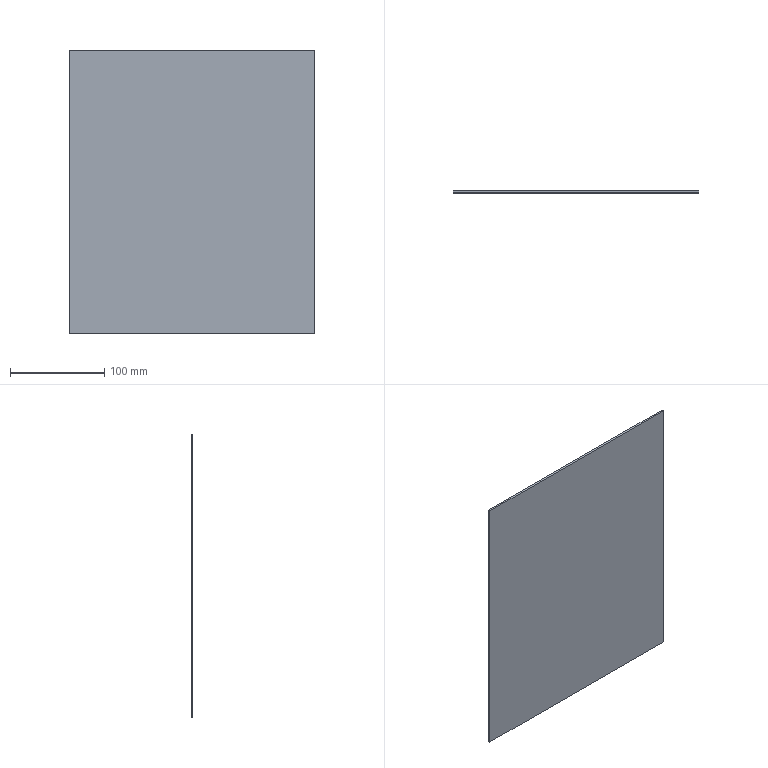Component | SolidWorks | SL010-Material-1 | 1 solid | 16 faces | box 260 x 2 x 300 mm | volume 155979 mm3 | plane 16
build123d program:
from build123d import *

# Parameters (mm, degrees)
SKETCH1_W           = 300
SKETCH1_H           = 260
BOSS_EXTRUDE1_DEPTH = 2
SKETCH2_W           = 284
SKETCH2_H           = 244
SKETCH2_W_2         = 283.6
SKETCH2_H_2         = 243.6
CUT_EXTRUDE1_DEPTH  = 0.1


with BuildPart() as part:
    # Sketch1 → Boss-Extrude1 (new body)
    with BuildSketch(Plane(origin=(0, 0, 0), x_dir=(1, 0, 0), z_dir=(0, 1, 0))):
        Rectangle(SKETCH1_W, SKETCH1_H)
    extrude(amount=BOSS_EXTRUDE1_DEPTH)

    # Sketch2 → Cut-Extrude1 (cut)
    with BuildSketch(Plane(origin=(0, 2, 0), x_dir=(1, 0, 0), z_dir=(0, 1, 0))):
        Rectangle(SKETCH2_W, SKETCH2_H)
        Rectangle(SKETCH2_W_2, SKETCH2_H_2, mode=Mode.SUBTRACT)
    extrude(amount=-CUT_EXTRUDE1_DEPTH, mode=Mode.SUBTRACT)


solid = part.part

# Placed as in the assembly
solid = solid.moved(Location((-535, -109.904, -487.035), (0, 90, 0)))
STEP:
#1=CARTESIAN_POINT('',(-15.945,-4.327,-25.08));
#2=VERTEX_POINT('',#1);
#3=CARTESIAN_POINT('',(-26.181,-4.327,-25.08));
#4=VERTEX_POINT('',#3);
#5=CARTESIAN_POINT('',(-26.181,-4.327,-25.08));
#6=DIRECTION('',(-1.,0.,0.));
#7=VECTOR('',#6,39.37);
#8=LINE('',#5,#7);
#9=EDGE_CURVE('',#2,#4,#8,.T.);
#10=ORIENTED_EDGE('',*,*,#9,.T.);
#11=CARTESIAN_POINT('',(-26.181,-4.248,-25.08));
#12=VERTEX_POINT('',#11);
#13=CARTESIAN_POINT('',(-26.181,-4.248,-25.08));
#14=DIRECTION('',(-0.,-1.,-0.));
#15=VECTOR('',#14,39.37);
#16=LINE('',#13,#15);
#17=EDGE_CURVE('',#12,#4,#16,.T.);
#18=ORIENTED_EDGE('',*,*,#17,.F.);
#19=CARTESIAN_POINT('',(-15.945,-4.248,-25.08));
#20=VERTEX_POINT('',#19);
#21=CARTESIAN_POINT('',(-26.181,-4.248,-25.08));
#22=DIRECTION('',(-1.,0.,0.));
#23=VECTOR('',#22,39.37);
#24=LINE('',#21,#23);
#25=EDGE_CURVE('',#20,#12,#24,.T.);
#26=ORIENTED_EDGE('',*,*,#25,.F.);
#27=CARTESIAN_POINT('',(-15.945,-4.248,-25.08));
#28=DIRECTION('',(-0.,-1.,-0.));
#29=VECTOR('',#28,39.37);
#30=LINE('',#27,#29);
#31=EDGE_CURVE('',#20,#2,#30,.T.);
#32=ORIENTED_EDGE('',*,*,#31,.T.);
#33=EDGE_LOOP('',(#10,#18,#26,#32));
#34=FACE_OUTER_BOUND('',#33,.T.);
#35=CARTESIAN_POINT('',(-26.181,-4.248,-25.08));
#36=DIRECTION('',(0.,-0.,1.));
#37=DIRECTION('',(1.,-0.,-0.));
#38=AXIS2_PLACEMENT_3D('',#35,#36,#37);
#39=PLANE('',#38);
#40=ADVANCED_FACE('',(#34),#39,.F.);
#41=CARTESIAN_POINT('',(-26.181,-4.327,-13.269));
#42=VERTEX_POINT('',#41);
#43=CARTESIAN_POINT('',(-26.181,-4.327,-13.269));
#44=DIRECTION('',(0.,-0.,1.));
#45=VECTOR('',#44,39.37);
#46=LINE('',#43,#45);
#47=EDGE_CURVE('',#4,#42,#46,.T.);
#48=ORIENTED_EDGE('',*,*,#47,.T.);
#49=CARTESIAN_POINT('',(-26.181,-4.248,-13.269));
#50=VERTEX_POINT('',#49);
#51=CARTESIAN_POINT('',(-26.181,-4.248,-13.269));
#52=DIRECTION('',(-0.,-1.,-0.));
#53=VECTOR('',#52,39.37);
#54=LINE('',#51,#53);
#55=EDGE_CURVE('',#50,#42,#54,.T.);
#56=ORIENTED_EDGE('',*,*,#55,.F.);
#57=CARTESIAN_POINT('',(-26.181,-4.248,-13.269));
#58=DIRECTION('',(0.,-0.,1.));
#59=VECTOR('',#58,39.37);
#60=LINE('',#57,#59);
#61=EDGE_CURVE('',#12,#50,#60,.T.);
#62=ORIENTED_EDGE('',*,*,#61,.F.);
#63=ORIENTED_EDGE('',*,*,#17,.T.);
#64=EDGE_LOOP('',(#48,#56,#62,#63));
#65=FACE_OUTER_BOUND('',#64,.T.);
#66=CARTESIAN_POINT('',(-26.181,-4.248,-13.269));
#67=DIRECTION('',(1.,-0.,-0.));
#68=DIRECTION('',(-0.,0.,-1.));
#69=AXIS2_PLACEMENT_3D('',#66,#67,#68);
#70=PLANE('',#69);
#71=ADVANCED_FACE('',(#65),#70,.F.);
#72=CARTESIAN_POINT('',(-15.945,-4.327,-13.269));
#73=VERTEX_POINT('',#72);
#74=CARTESIAN_POINT('',(-26.181,-4.327,-13.269));
#75=DIRECTION('',(1.,-0.,-0.));
#76=VECTOR('',#75,39.37);
#77=LINE('',#74,#76);
#78=EDGE_CURVE('',#42,#73,#77,.T.);
#79=ORIENTED_EDGE('',*,*,#78,.T.);
#80=CARTESIAN_POINT('',(-15.945,-4.248,-13.269));
#81=VERTEX_POINT('',#80);
#82=CARTESIAN_POINT('',(-15.945,-4.248,-13.269));
#83=DIRECTION('',(-0.,-1.,-0.));
#84=VECTOR('',#83,39.37);
#85=LINE('',#82,#84);
#86=EDGE_CURVE('',#81,#73,#85,.T.);
#87=ORIENTED_EDGE('',*,*,#86,.F.);
#88=CARTESIAN_POINT('',(-26.181,-4.248,-13.269));
#89=DIRECTION('',(1.,-0.,-0.));
#90=VECTOR('',#89,39.37);
#91=LINE('',#88,#90);
#92=EDGE_CURVE('',#50,#81,#91,.T.);
#93=ORIENTED_EDGE('',*,*,#92,.F.);
#94=ORIENTED_EDGE('',*,*,#55,.T.);
#95=EDGE_LOOP('',(#79,#87,#93,#94));
#96=FACE_OUTER_BOUND('',#95,.T.);
#97=CARTESIAN_POINT('',(-26.181,-4.248,-13.269));
#98=DIRECTION('',(-0.,0.,-1.));
#99=DIRECTION('',(-1.,0.,0.));
#100=AXIS2_PLACEMENT_3D('',#97,#98,#99);
#101=PLANE('',#100);
#102=ADVANCED_FACE('',(#96),#101,.F.);
#103=CARTESIAN_POINT('',(-15.945,-4.327,-13.269));
#104=DIRECTION('',(-0.,0.,-1.));
#105=VECTOR('',#104,39.37);
#106=LINE('',#103,#105);
#107=EDGE_CURVE('',#73,#2,#106,.T.);
#108=ORIENTED_EDGE('',*,*,#107,.T.);
#109=ORIENTED_EDGE('',*,*,#31,.F.);
#110=CARTESIAN_POINT('',(-15.945,-4.248,-13.269));
#111=DIRECTION('',(-0.,0.,-1.));
#112=VECTOR('',#111,39.37);
#113=LINE('',#110,#112);
#114=EDGE_CURVE('',#81,#20,#113,.T.);
#115=ORIENTED_EDGE('',*,*,#114,.F.);
#116=ORIENTED_EDGE('',*,*,#86,.T.);
#117=EDGE_LOOP('',(#108,#109,#115,#116));
#118=FACE_OUTER_BOUND('',#117,.T.);
#119=CARTESIAN_POINT('',(-15.945,-4.248,-13.269));
#120=DIRECTION('',(-1.,0.,0.));
#121=DIRECTION('',(0.,-0.,1.));
#122=AXIS2_PLACEMENT_3D('',#119,#120,#121);
#123=PLANE('',#122);
#124=ADVANCED_FACE('',(#118),#123,.F.);
#125=CARTESIAN_POINT('',(-16.26,-4.248,-13.584));
#126=VERTEX_POINT('',#125);
#127=CARTESIAN_POINT('',(-16.26,-4.248,-24.765));
#128=VERTEX_POINT('',#127);
#129=CARTESIAN_POINT('',(-16.26,-4.248,-13.584));
#130=DIRECTION('',(-0.,0.,-1.));
#131=VECTOR('',#130,39.37);
#132=LINE('',#129,#131);
#133=EDGE_CURVE('',#126,#128,#132,.T.);
#134=ORIENTED_EDGE('',*,*,#133,.F.);
#135=CARTESIAN_POINT('',(-25.866,-4.248,-13.584));
#136=VERTEX_POINT('',#135);
#137=CARTESIAN_POINT('',(-25.866,-4.248,-13.584));
#138=DIRECTION('',(1.,-0.,-0.));
#139=VECTOR('',#138,39.37);
#140=LINE('',#137,#139);
#141=EDGE_CURVE('',#136,#126,#140,.T.);
#142=ORIENTED_EDGE('',*,*,#141,.F.);
#143=CARTESIAN_POINT('',(-25.866,-4.248,-24.765));
#144=VERTEX_POINT('',#143);
#145=CARTESIAN_POINT('',(-25.866,-4.248,-24.765));
#146=DIRECTION('',(0.,-0.,1.));
#147=VECTOR('',#146,39.37);
#148=LINE('',#145,#147);
#149=EDGE_CURVE('',#144,#136,#148,.T.);
#150=ORIENTED_EDGE('',*,*,#149,.F.);
#151=CARTESIAN_POINT('',(-16.26,-4.248,-24.765));
#152=DIRECTION('',(-1.,0.,0.));
#153=VECTOR('',#152,39.37);
#154=LINE('',#151,#153);
#155=EDGE_CURVE('',#128,#144,#154,.T.);
#156=ORIENTED_EDGE('',*,*,#155,.F.);
#157=EDGE_LOOP('',(#134,#142,#150,#156));
#158=FACE_BOUND('',#157,.T.);
#159=ORIENTED_EDGE('',*,*,#25,.T.);
#160=ORIENTED_EDGE('',*,*,#61,.T.);
#161=ORIENTED_EDGE('',*,*,#92,.T.);
#162=ORIENTED_EDGE('',*,*,#114,.T.);
#163=EDGE_LOOP('',(#159,#160,#161,#162));
#164=FACE_OUTER_BOUND('',#163,.T.);
#165=CARTESIAN_POINT('',(-21.063,-4.248,-19.175));
#166=DIRECTION('',(0.,1.,0.));
#167=DIRECTION('',(1.,-0.,-0.));
#168=AXIS2_PLACEMENT_3D('',#165,#166,#167);
#169=PLANE('',#168);
#170=ADVANCED_FACE('',(#158,#164),#169,.T.);
#171=ORIENTED_EDGE('',*,*,#9,.F.);
#172=ORIENTED_EDGE('',*,*,#107,.F.);
#173=ORIENTED_EDGE('',*,*,#78,.F.);
#174=ORIENTED_EDGE('',*,*,#47,.F.);
#175=EDGE_LOOP('',(#171,#172,#173,#174));
#176=FACE_OUTER_BOUND('',#175,.T.);
#177=CARTESIAN_POINT('',(-21.063,-4.327,-19.175));
#178=DIRECTION('',(0.,1.,0.));
#179=DIRECTION('',(1.,-0.,-0.));
#180=AXIS2_PLACEMENT_3D('',#177,#178,#179);
#181=PLANE('',#180);
#182=ADVANCED_FACE('',(#176),#181,.F.);
#183=ORIENTED_EDGE('',*,*,#133,.T.);
#184=CARTESIAN_POINT('',(-16.26,-4.252,-24.765));
#185=VERTEX_POINT('',#184);
#186=CARTESIAN_POINT('',(-16.26,-4.252,-24.765));
#187=DIRECTION('',(0.,1.,0.));
#188=VECTOR('',#187,39.37);
#189=LINE('',#186,#188);
#190=EDGE_CURVE('',#185,#128,#189,.T.);
#191=ORIENTED_EDGE('',*,*,#190,.F.);
#192=CARTESIAN_POINT('',(-16.26,-4.252,-13.584));
#193=VERTEX_POINT('',#192);
#194=CARTESIAN_POINT('',(-16.26,-4.252,-13.584));
#195=DIRECTION('',(-0.,0.,-1.));
#196=VECTOR('',#195,39.37);
#197=LINE('',#194,#196);
#198=EDGE_CURVE('',#193,#185,#197,.T.);
#199=ORIENTED_EDGE('',*,*,#198,.F.);
#200=CARTESIAN_POINT('',(-16.26,-4.252,-13.584));
#201=DIRECTION('',(0.,1.,0.));
#202=VECTOR('',#201,39.37);
#203=LINE('',#200,#202);
#204=EDGE_CURVE('',#193,#126,#203,.T.);
#205=ORIENTED_EDGE('',*,*,#204,.T.);
#206=EDGE_LOOP('',(#183,#191,#199,#205));
#207=FACE_OUTER_BOUND('',#206,.T.);
#208=CARTESIAN_POINT('',(-16.26,-4.252,-13.584));
#209=DIRECTION('',(1.,-0.,-0.));
#210=DIRECTION('',(-0.,0.,-1.));
#211=AXIS2_PLACEMENT_3D('',#208,#209,#210);
#212=PLANE('',#211);
#213=ADVANCED_FACE('',(#207),#212,.F.);
#214=ORIENTED_EDGE('',*,*,#141,.T.);
#215=ORIENTED_EDGE('',*,*,#204,.F.);
#216=CARTESIAN_POINT('',(-25.866,-4.252,-13.584));
#217=VERTEX_POINT('',#216);
#218=CARTESIAN_POINT('',(-25.866,-4.252,-13.584));
#219=DIRECTION('',(1.,-0.,-0.));
#220=VECTOR('',#219,39.37);
#221=LINE('',#218,#220);
#222=EDGE_CURVE('',#217,#193,#221,.T.);
#223=ORIENTED_EDGE('',*,*,#222,.F.);
#224=CARTESIAN_POINT('',(-25.866,-4.252,-13.584));
#225=DIRECTION('',(0.,1.,0.));
#226=VECTOR('',#225,39.37);
#227=LINE('',#224,#226);
#228=EDGE_CURVE('',#217,#136,#227,.T.);
#229=ORIENTED_EDGE('',*,*,#228,.T.);
#230=EDGE_LOOP('',(#214,#215,#223,#229));
#231=FACE_OUTER_BOUND('',#230,.T.);
#232=CARTESIAN_POINT('',(-25.866,-4.252,-13.584));
#233=DIRECTION('',(0.,-0.,1.));
#234=DIRECTION('',(1.,-0.,-0.));
#235=AXIS2_PLACEMENT_3D('',#232,#233,#234);
#236=PLANE('',#235);
#237=ADVANCED_FACE('',(#231),#236,.F.);
#238=ORIENTED_EDGE('',*,*,#149,.T.);
#239=ORIENTED_EDGE('',*,*,#228,.F.);
#240=CARTESIAN_POINT('',(-25.866,-4.252,-24.765));
#241=VERTEX_POINT('',#240);
#242=CARTESIAN_POINT('',(-25.866,-4.252,-24.765));
#243=DIRECTION('',(0.,-0.,1.));
#244=VECTOR('',#243,39.37);
#245=LINE('',#242,#244);
#246=EDGE_CURVE('',#241,#217,#245,.T.);
#247=ORIENTED_EDGE('',*,*,#246,.F.);
#248=CARTESIAN_POINT('',(-25.866,-4.252,-24.765));
#249=DIRECTION('',(0.,1.,0.));
#250=VECTOR('',#249,39.37);
#251=LINE('',#248,#250);
#252=EDGE_CURVE('',#241,#144,#251,.T.);
#253=ORIENTED_EDGE('',*,*,#252,.T.);
#254=EDGE_LOOP('',(#238,#239,#247,#253));
#255=FACE_OUTER_BOUND('',#254,.T.);
#256=CARTESIAN_POINT('',(-25.866,-4.252,-24.765));
#257=DIRECTION('',(-1.,0.,0.));
#258=DIRECTION('',(0.,-0.,1.));
#259=AXIS2_PLACEMENT_3D('',#256,#257,#258);
#260=PLANE('',#259);
#261=ADVANCED_FACE('',(#255),#260,.F.);
#262=ORIENTED_EDGE('',*,*,#155,.T.);
#263=ORIENTED_EDGE('',*,*,#252,.F.);
#264=CARTESIAN_POINT('',(-16.26,-4.252,-24.765));
#265=DIRECTION('',(-1.,0.,0.));
#266=VECTOR('',#265,39.37);
#267=LINE('',#264,#266);
#268=EDGE_CURVE('',#185,#241,#267,.T.);
#269=ORIENTED_EDGE('',*,*,#268,.F.);
#270=ORIENTED_EDGE('',*,*,#190,.T.);
#271=EDGE_LOOP('',(#262,#263,#269,#270));
#272=FACE_OUTER_BOUND('',#271,.T.);
#273=CARTESIAN_POINT('',(-16.26,-4.252,-24.765));
#274=DIRECTION('',(-0.,0.,-1.));
#275=DIRECTION('',(-1.,0.,0.));
#276=AXIS2_PLACEMENT_3D('',#273,#274,#275);
#277=PLANE('',#276);
#278=ADVANCED_FACE('',(#272),#277,.F.);
#279=CARTESIAN_POINT('',(-25.858,-4.252,-13.592));
#280=VERTEX_POINT('',#279);
#281=CARTESIAN_POINT('',(-16.268,-4.252,-13.592));
#282=VERTEX_POINT('',#281);
#283=CARTESIAN_POINT('',(-25.858,-4.252,-13.592));
#284=DIRECTION('',(1.,-0.,-0.));
#285=VECTOR('',#284,39.37);
#286=LINE('',#283,#285);
#287=EDGE_CURVE('',#280,#282,#286,.T.);
#288=ORIENTED_EDGE('',*,*,#287,.F.);
#289=CARTESIAN_POINT('',(-25.858,-4.252,-24.757));
#290=VERTEX_POINT('',#289);
#291=CARTESIAN_POINT('',(-25.858,-4.252,-24.757));
#292=DIRECTION('',(0.,-0.,1.));
#293=VECTOR('',#292,39.37);
#294=LINE('',#291,#293);
#295=EDGE_CURVE('',#290,#280,#294,.T.);
#296=ORIENTED_EDGE('',*,*,#295,.F.);
#297=CARTESIAN_POINT('',(-16.268,-4.252,-24.757));
#298=VERTEX_POINT('',#297);
#299=CARTESIAN_POINT('',(-16.268,-4.252,-24.757));
#300=DIRECTION('',(-1.,0.,0.));
#301=VECTOR('',#300,39.37);
#302=LINE('',#299,#301);
#303=EDGE_CURVE('',#298,#290,#302,.T.);
#304=ORIENTED_EDGE('',*,*,#303,.F.);
#305=CARTESIAN_POINT('',(-16.268,-4.252,-13.592));
#306=DIRECTION('',(-0.,0.,-1.));
#307=VECTOR('',#306,39.37);
#308=LINE('',#305,#307);
#309=EDGE_CURVE('',#282,#298,#308,.T.);
#310=ORIENTED_EDGE('',*,*,#309,.F.);
#311=EDGE_LOOP('',(#288,#296,#304,#310));
#312=FACE_BOUND('',#311,.T.);
#313=ORIENTED_EDGE('',*,*,#198,.T.);
#314=ORIENTED_EDGE('',*,*,#268,.T.);
#315=ORIENTED_EDGE('',*,*,#246,.T.);
#316=ORIENTED_EDGE('',*,*,#222,.T.);
#317=EDGE_LOOP('',(#313,#314,#315,#316));
#318=FACE_OUTER_BOUND('',#317,.T.);
#319=CARTESIAN_POINT('',(-21.063,-4.252,-19.175));
#320=DIRECTION('',(0.,1.,0.));
#321=DIRECTION('',(1.,-0.,-0.));
#322=AXIS2_PLACEMENT_3D('',#319,#320,#321);
#323=PLANE('',#322);
#324=ADVANCED_FACE('',(#312,#318),#323,.T.);
#325=CARTESIAN_POINT('',(-16.268,-4.248,-13.592));
#326=VERTEX_POINT('',#325);
#327=CARTESIAN_POINT('',(-16.268,-4.248,-24.757));
#328=VERTEX_POINT('',#327);
#329=CARTESIAN_POINT('',(-16.268,-4.248,-13.592));
#330=DIRECTION('',(-0.,0.,-1.));
#331=VECTOR('',#330,39.37);
#332=LINE('',#329,#331);
#333=EDGE_CURVE('',#326,#328,#332,.T.);
#334=ORIENTED_EDGE('',*,*,#333,.F.);
#335=CARTESIAN_POINT('',(-16.268,-4.252,-13.592));
#336=DIRECTION('',(0.,1.,0.));
#337=VECTOR('',#336,39.37);
#338=LINE('',#335,#337);
#339=EDGE_CURVE('',#282,#326,#338,.T.);
#340=ORIENTED_EDGE('',*,*,#339,.F.);
#341=ORIENTED_EDGE('',*,*,#309,.T.);
#342=CARTESIAN_POINT('',(-16.268,-4.252,-24.757));
#343=DIRECTION('',(0.,1.,0.));
#344=VECTOR('',#343,39.37);
#345=LINE('',#342,#344);
#346=EDGE_CURVE('',#298,#328,#345,.T.);
#347=ORIENTED_EDGE('',*,*,#346,.T.);
#348=EDGE_LOOP('',(#334,#340,#341,#347));
#349=FACE_OUTER_BOUND('',#348,.T.);
#350=CARTESIAN_POINT('',(-16.268,-4.252,-13.592));
#351=DIRECTION('',(1.,-0.,-0.));
#352=DIRECTION('',(-0.,0.,-1.));
#353=AXIS2_PLACEMENT_3D('',#350,#351,#352);
#354=PLANE('',#353);
#355=ADVANCED_FACE('',(#349),#354,.T.);
#356=CARTESIAN_POINT('',(-25.858,-4.248,-13.592));
#357=VERTEX_POINT('',#356);
#358=CARTESIAN_POINT('',(-25.858,-4.248,-13.592));
#359=DIRECTION('',(1.,-0.,-0.));
#360=VECTOR('',#359,39.37);
#361=LINE('',#358,#360);
#362=EDGE_CURVE('',#357,#326,#361,.T.);
#363=ORIENTED_EDGE('',*,*,#362,.F.);
#364=CARTESIAN_POINT('',(-25.858,-4.252,-13.592));
#365=DIRECTION('',(0.,1.,0.));
#366=VECTOR('',#365,39.37);
#367=LINE('',#364,#366);
#368=EDGE_CURVE('',#280,#357,#367,.T.);
#369=ORIENTED_EDGE('',*,*,#368,.F.);
#370=ORIENTED_EDGE('',*,*,#287,.T.);
#371=ORIENTED_EDGE('',*,*,#339,.T.);
#372=EDGE_LOOP('',(#363,#369,#370,#371));
#373=FACE_OUTER_BOUND('',#372,.T.);
#374=CARTESIAN_POINT('',(-25.858,-4.252,-13.592));
#375=DIRECTION('',(0.,-0.,1.));
#376=DIRECTION('',(1.,-0.,-0.));
#377=AXIS2_PLACEMENT_3D('',#374,#375,#376);
#378=PLANE('',#377);
#379=ADVANCED_FACE('',(#373),#378,.T.);
#380=CARTESIAN_POINT('',(-25.858,-4.248,-24.757));
#381=VERTEX_POINT('',#380);
#382=CARTESIAN_POINT('',(-25.858,-4.248,-24.757));
#383=DIRECTION('',(0.,-0.,1.));
#384=VECTOR('',#383,39.37);
#385=LINE('',#382,#384);
#386=EDGE_CURVE('',#381,#357,#385,.T.);
#387=ORIENTED_EDGE('',*,*,#386,.F.);
#388=CARTESIAN_POINT('',(-25.858,-4.252,-24.757));
#389=DIRECTION('',(0.,1.,0.));
#390=VECTOR('',#389,39.37);
#391=LINE('',#388,#390);
#392=EDGE_CURVE('',#290,#381,#391,.T.);
#393=ORIENTED_EDGE('',*,*,#392,.F.);
#394=ORIENTED_EDGE('',*,*,#295,.T.);
#395=ORIENTED_EDGE('',*,*,#368,.T.);
#396=EDGE_LOOP('',(#387,#393,#394,#395));
#397=FACE_OUTER_BOUND('',#396,.T.);
#398=CARTESIAN_POINT('',(-25.858,-4.252,-24.757));
#399=DIRECTION('',(-1.,0.,0.));
#400=DIRECTION('',(0.,-0.,1.));
#401=AXIS2_PLACEMENT_3D('',#398,#399,#400);
#402=PLANE('',#401);
#403=ADVANCED_FACE('',(#397),#402,.T.);
#404=CARTESIAN_POINT('',(-16.268,-4.248,-24.757));
#405=DIRECTION('',(-1.,0.,0.));
#406=VECTOR('',#405,39.37);
#407=LINE('',#404,#406);
#408=EDGE_CURVE('',#328,#381,#407,.T.);
#409=ORIENTED_EDGE('',*,*,#408,.F.);
#410=ORIENTED_EDGE('',*,*,#346,.F.);
#411=ORIENTED_EDGE('',*,*,#303,.T.);
#412=ORIENTED_EDGE('',*,*,#392,.T.);
#413=EDGE_LOOP('',(#409,#410,#411,#412));
#414=FACE_OUTER_BOUND('',#413,.T.);
#415=CARTESIAN_POINT('',(-16.268,-4.252,-24.757));
#416=DIRECTION('',(-0.,0.,-1.));
#417=DIRECTION('',(-1.,0.,0.));
#418=AXIS2_PLACEMENT_3D('',#415,#416,#417);
#419=PLANE('',#418);
#420=ADVANCED_FACE('',(#414),#419,.T.);
#421=ORIENTED_EDGE('',*,*,#362,.T.);
#422=ORIENTED_EDGE('',*,*,#333,.T.);
#423=ORIENTED_EDGE('',*,*,#408,.T.);
#424=ORIENTED_EDGE('',*,*,#386,.T.);
#425=EDGE_LOOP('',(#421,#422,#423,#424));
#426=FACE_OUTER_BOUND('',#425,.T.);
#427=CARTESIAN_POINT('',(-21.063,-4.248,-19.175));
#428=DIRECTION('',(0.,1.,0.));
#429=DIRECTION('',(1.,-0.,-0.));
#430=AXIS2_PLACEMENT_3D('',#427,#428,#429);
#431=PLANE('',#430);
#432=ADVANCED_FACE('',(#426),#431,.T.);
#433=CLOSED_SHELL('',(#40,#71,#102,#124,#170,#182,#213,#237,#261,#278,#324,#355,#379,#403,#420,#432));
#434=MANIFOLD_SOLID_BREP('',#433);
#435=CARTESIAN_POINT('',(0.,0.,0.));
#436=DIRECTION('',(0.,0.,1.));
#437=DIRECTION('',(1.,0.,0.));
#438=AXIS2_PLACEMENT_3D('',#435,#436,#437);
#439=(LENGTH_UNIT()NAMED_UNIT(*)SI_UNIT($,.METRE.));
#440=LENGTH_MEASURE_WITH_UNIT(LENGTH_MEASURE(0.0254),#439);
#441=DIMENSIONAL_EXPONENTS(1.,0.,0.,0.,0.,0.,0.);
#442=(CONVERSION_BASED_UNIT('',#440)LENGTH_UNIT()NAMED_UNIT(#441));
#443=UNCERTAINTY_MEASURE_WITH_UNIT(LENGTH_MEASURE(0.00001),#442,'','');
#444=(NAMED_UNIT(*)PLANE_ANGLE_UNIT()SI_UNIT($,.RADIAN.));
#445=(NAMED_UNIT(*)SI_UNIT($,.STERADIAN.)SOLID_ANGLE_UNIT());
#446=(GEOMETRIC_REPRESENTATION_CONTEXT(3)GLOBAL_UNCERTAINTY_ASSIGNED_CONTEXT((#443))GLOBAL_UNIT_ASSIGNED_CONTEXT((#442,#444,#445))REPRESENTATION_CONTEXT('',''));
#447=ADVANCED_BREP_SHAPE_REPRESENTATION('',(#434,#438),#446);
#448=COLOUR_RGB('',0.7922,0.8196,0.9333);
#449=FILL_AREA_STYLE_COLOUR('',#448);
#450=FILL_AREA_STYLE('',(#449));
#451=SURFACE_STYLE_FILL_AREA(#450);
#452=SURFACE_SIDE_STYLE('',(#451));
#453=SURFACE_STYLE_USAGE(.BOTH.,#452);
#454=PRESENTATION_STYLE_ASSIGNMENT((#453));
#455=STYLED_ITEM('',(#454),#434);
#456=(LENGTH_UNIT()NAMED_UNIT(*)SI_UNIT($,.METRE.));
#457=LENGTH_MEASURE_WITH_UNIT(LENGTH_MEASURE(0.0254),#456);
#458=DIMENSIONAL_EXPONENTS(1.,0.,0.,0.,0.,0.,0.);
#459=(CONVERSION_BASED_UNIT('',#457)LENGTH_UNIT()NAMED_UNIT(#458));
#460=UNCERTAINTY_MEASURE_WITH_UNIT(LENGTH_MEASURE(0.00001),#459,'','');
#461=(NAMED_UNIT(*)PLANE_ANGLE_UNIT()SI_UNIT($,.RADIAN.));
#462=(NAMED_UNIT(*)SI_UNIT($,.STERADIAN.)SOLID_ANGLE_UNIT());
#463=(GEOMETRIC_REPRESENTATION_CONTEXT(3)GLOBAL_UNCERTAINTY_ASSIGNED_CONTEXT((#460))GLOBAL_UNIT_ASSIGNED_CONTEXT((#459,#461,#462))REPRESENTATION_CONTEXT('',''));
#464=MECHANICAL_DESIGN_GEOMETRIC_PRESENTATION_REPRESENTATION('',(#455),#463);
#465=PRESENTATION_LAYER_ASSIGNMENT('','',(#455));